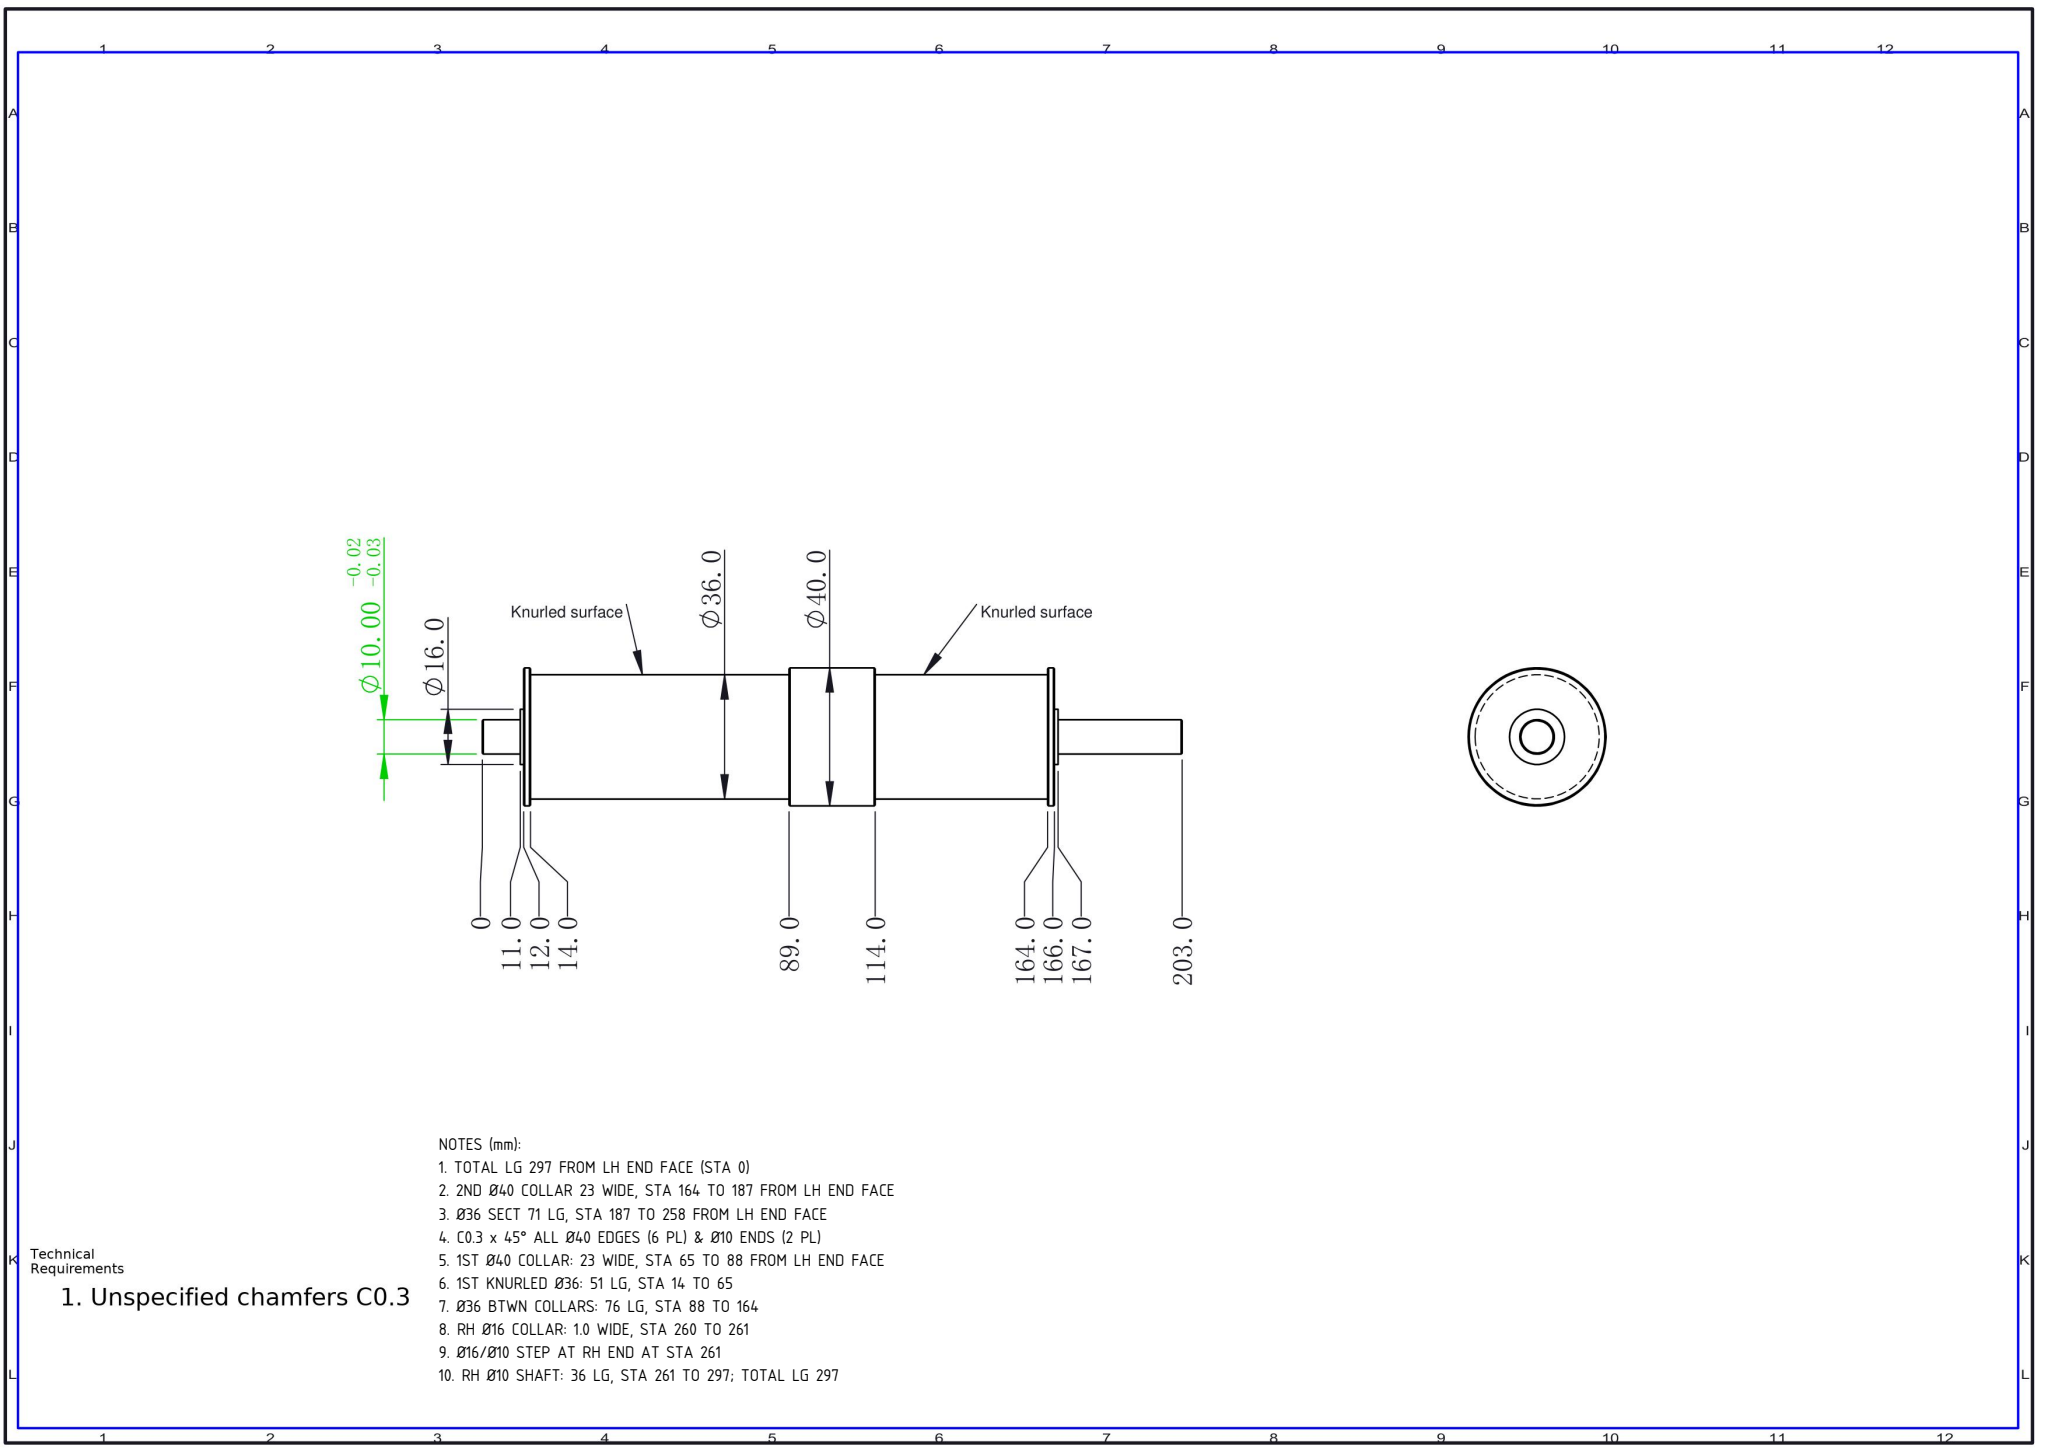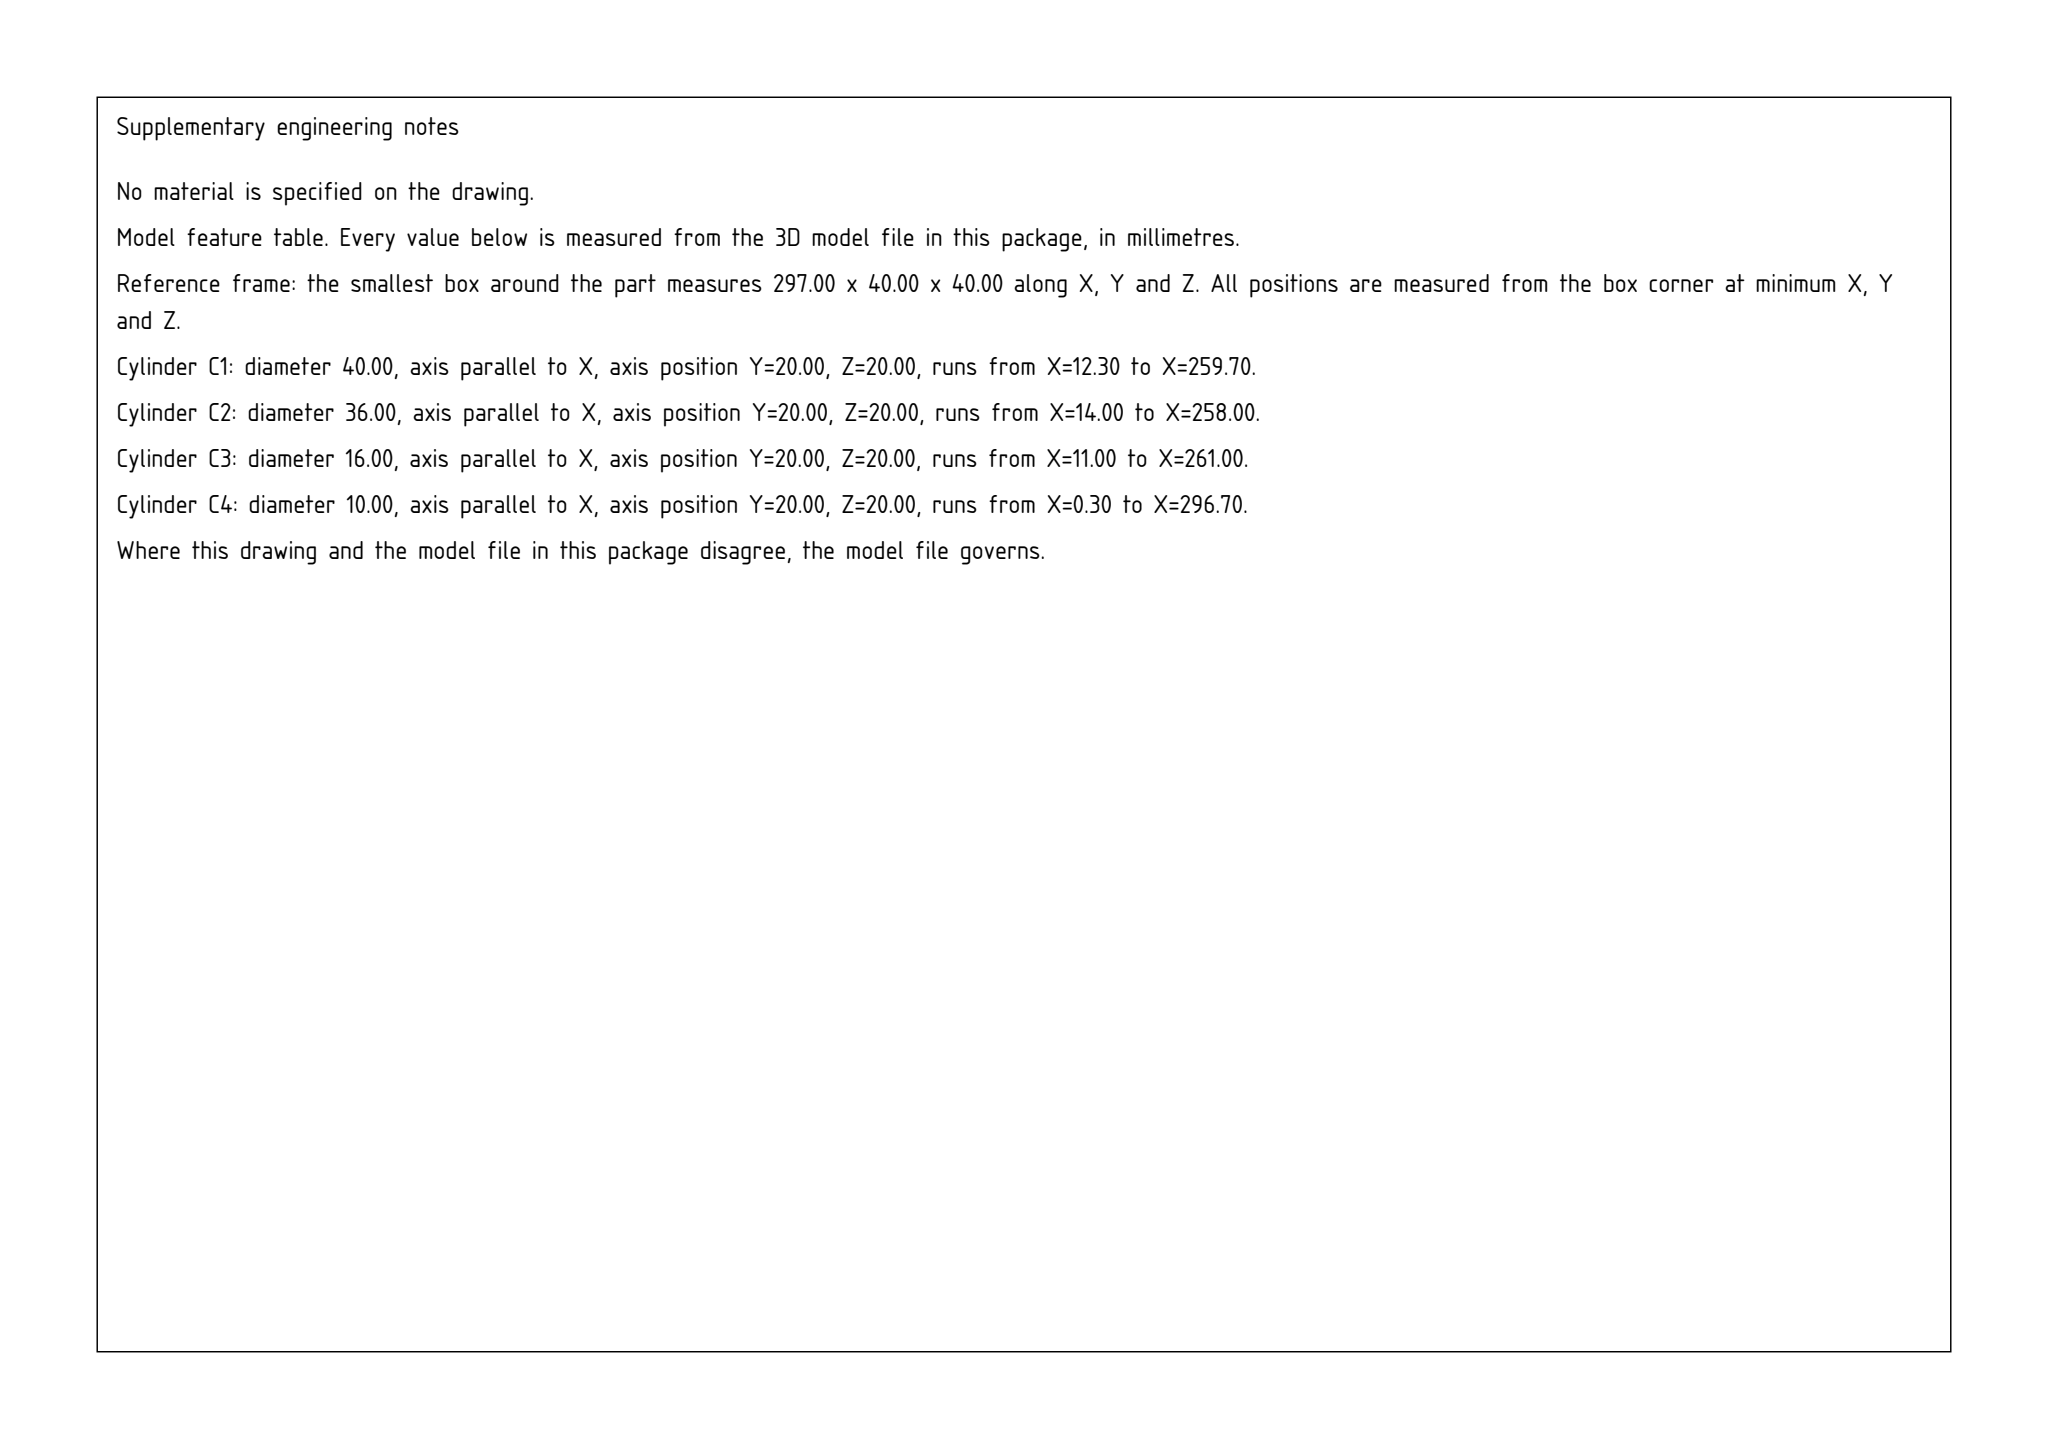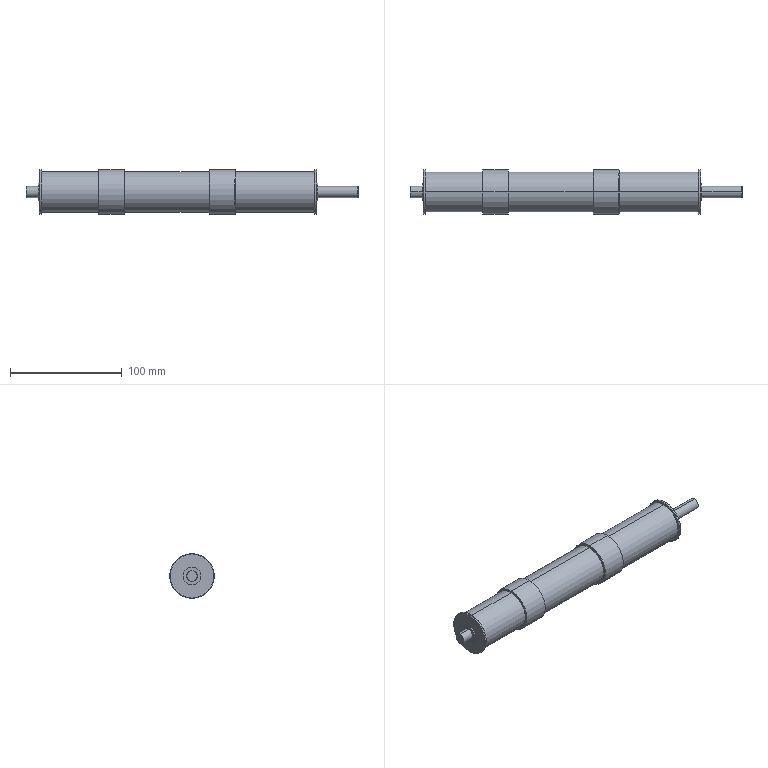Part | SolidWorks | mm | 1 solid | 50 faces | box 297 x 40 x 40 mm | volume 268428 mm3 | cylinder 22 | cone 16 | plane 12 | commonest cylinder face diameters 40 x8 36 x6 10 x4 16 x4
Drawing notes:
TOTAL LG 297 FROM LH END FACE (STA 0) | from the solid: bbox_xyz x = 297.0; x-planes 0.0 and 297.0
2ND Ø40 COLLAR 23 WIDE, STA 164 TO 187 FROM LH END FACE | from the solid: cyl dia40 len23 on x; x-planes 164.0 and 187.0
Ø36 SECT 71 LG, STA 187 TO 258 FROM LH END FACE | from the solid: cyl dia36 len71; x-planes 187.0 and 258.0
C0.3 x 45° ALL Ø40 EDGES (6 PL) & Ø10 ENDS (2 PL) | from the solid: cones 90° incl, ref dia 39.4/40.0 (6) and 9.4/10.0 (2)
1ST Ø40 COLLAR: 23 WIDE, STA 65 TO 88 FROM LH END FACE | from the solid: Ø40 cyl L=23 between x-planes 65 and 88 (22.4 + 2x C0.3)
1ST KNURLED Ø36: 51 LG, STA 14 TO 65 | from the solid: Ø36 cyl L=51 between x-planes 14 and 65
Ø36 BTWN COLLARS: 76 LG, STA 88 TO 164 | from the solid: Ø36 cyl L=76 between x-planes 88 and 164
RH Ø16 COLLAR: 1.0 WIDE, STA 260 TO 261 | from the solid: Ø16 cyl L=1.0 between x-planes 260 and 261
Ø16/Ø10 STEP AT RH END AT STA 261 | from the solid: x-plane 261 = end of Ø16, start of Ø10 cyl
RH Ø10 SHAFT: 36 LG, STA 261 TO 297; TOTAL LG 297 | from the solid: Ø10 cyl L=35.7+C0.3 from x=261 to bbox 297
build123d program:
from build123d import *

# Parameters (mm, degrees)
CHAMFER1_SIZE = 0.3


with BuildPart() as part:
    # Sketch1 → Revolve1 (revolve)
    with BuildSketch(Plane.XY, mode=Mode.PRIVATE) as revolve1_sk:
        Polygon((258, 20), (260, 20), (260, 8), (261, 8), (261, 5), (297, 5), (297, 0), (0, 0), (0, 5), (11, 5), (11, 8), (12, 8), (12, 20), (14, 20), (14, 18), (65, 18), (65, 20), (88, 20), (88, 18), (164, 18), (164, 20), (187, 20), (187, 18), (258, 18), align=None)
    revolve(revolve1_sk.sketch.rotate(Axis((0, 0, 0), (1, 0, 0)), 90), axis=Axis((0, 0, 0), (1, 0, 0)))

    # Chamfer1
    chamfer1_edges = [part.edges().sort_by_distance(p)[0] for p in [
        (297, 0, -5),
        (260, 0, -20),
        (258, 0, -20),
        (187, 0, -20),
        (164, 0, -20),
        (14, 0, -20),
        (12, 0, -20),
        (0, 0, -5),
    ]]
    chamfer(chamfer1_edges, length=CHAMFER1_SIZE)


solid = part.part